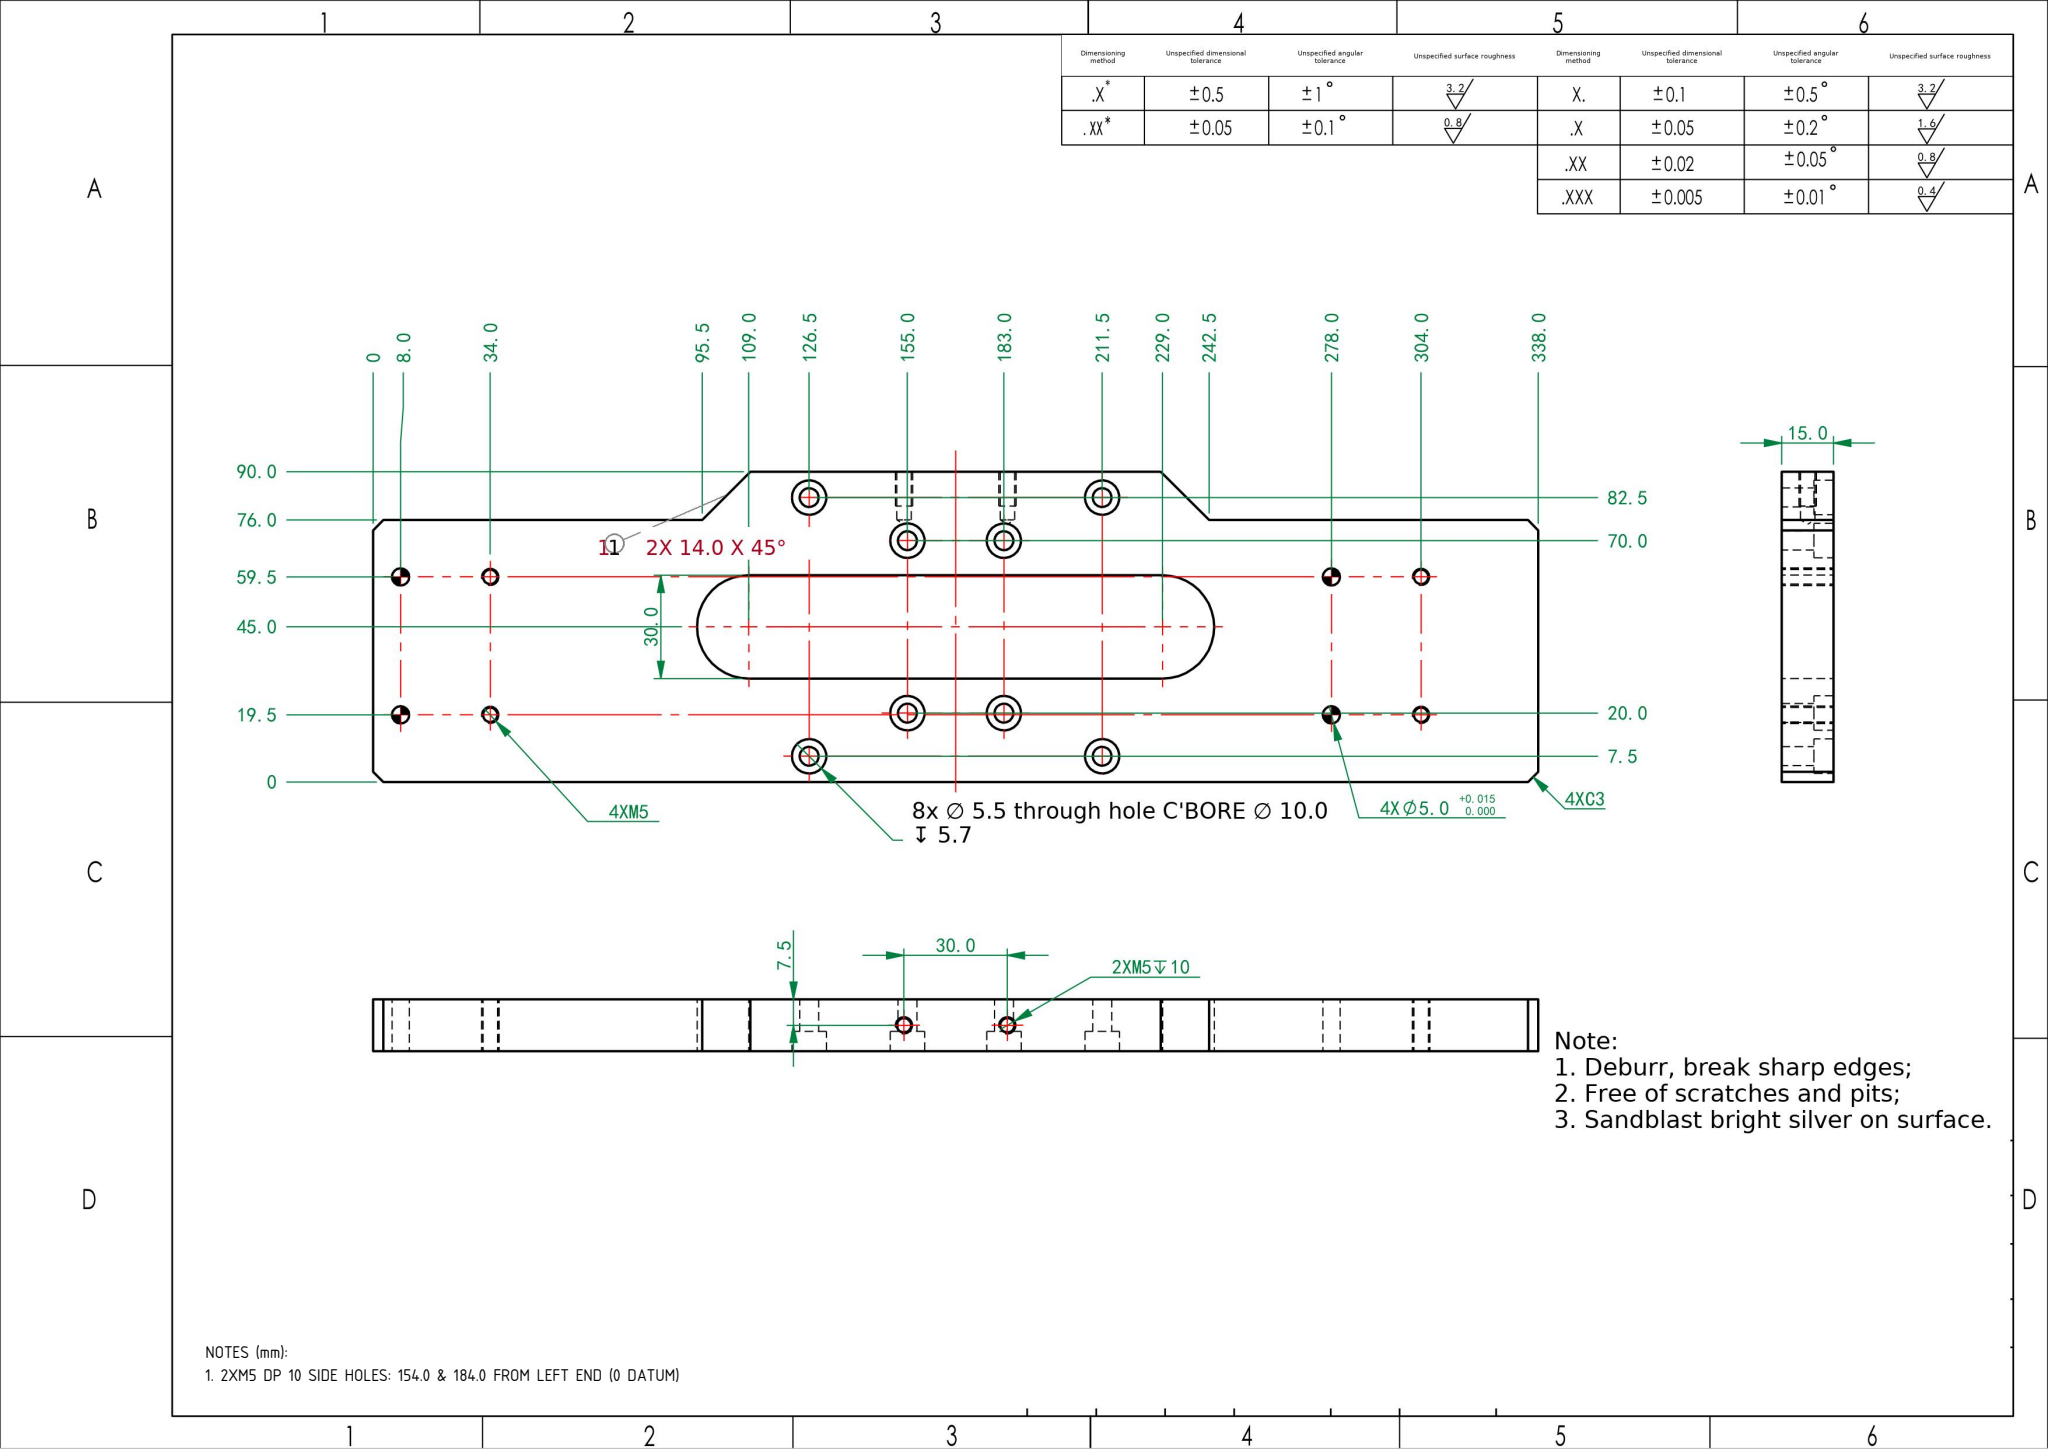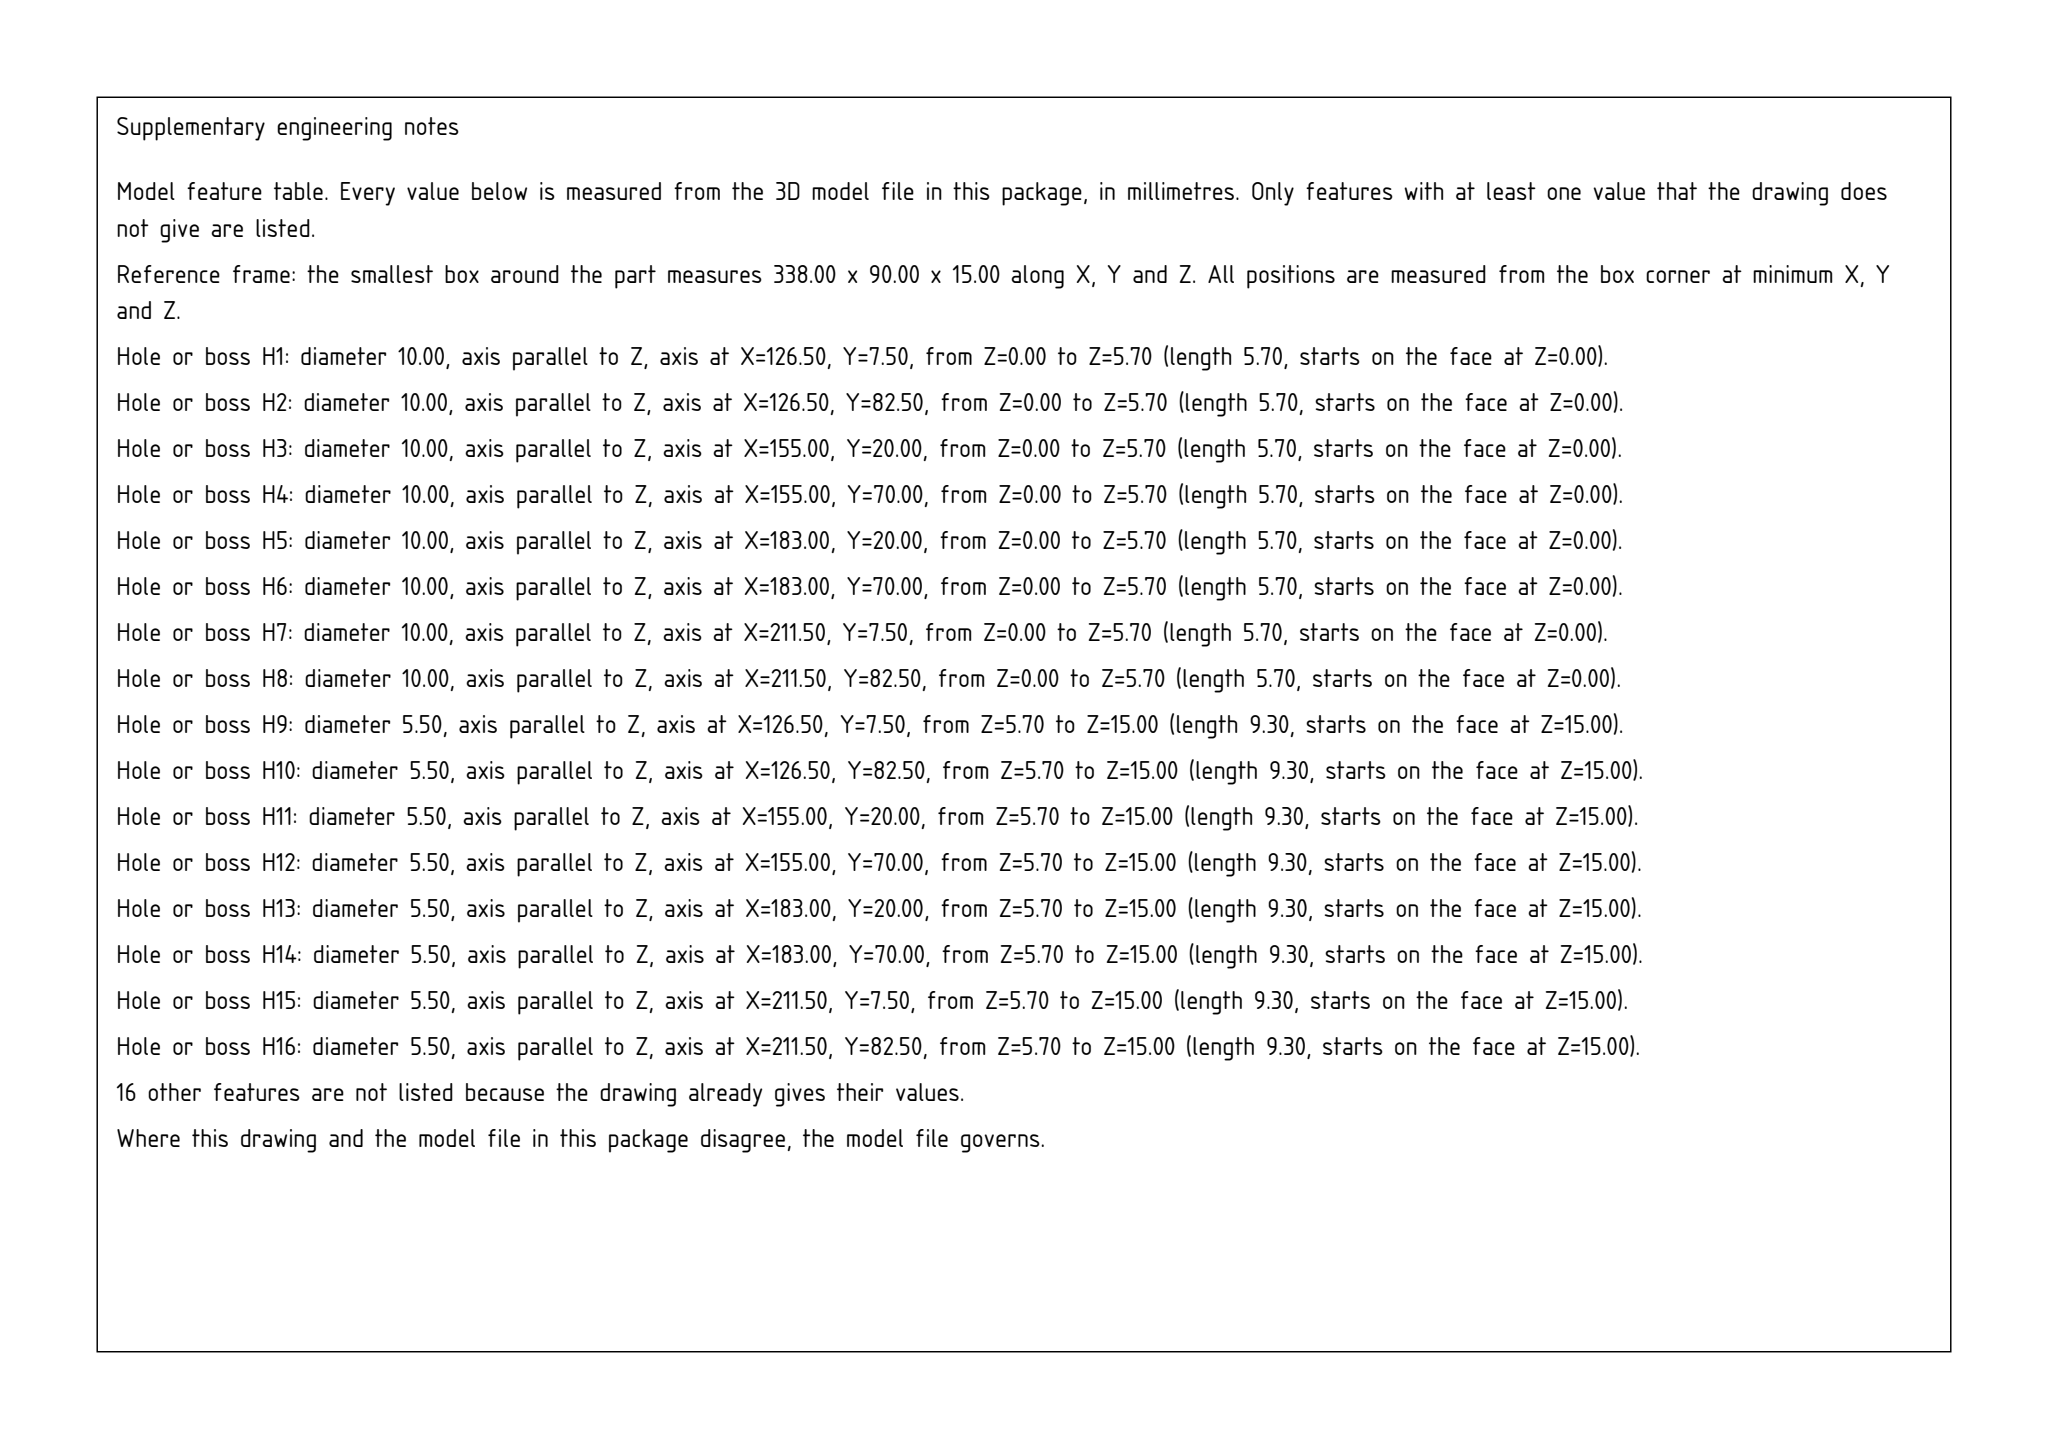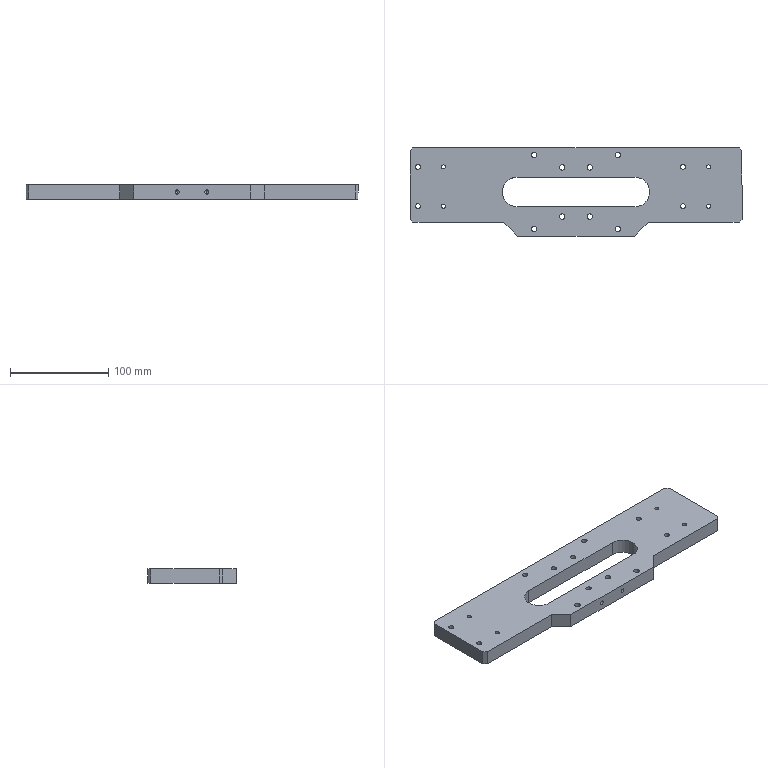Part | SolidWorks | mm | 1 solid | 83 faces | box 338 x 90 x 15 mm | volume 340619 mm3 | cylinder 55 | plane 24 | cone 4 | commonest cylinder face diameters 10 x16 5.5 x16 4.2 x12 5 x8 30 x3
Drawing notes:
2XM5 DP 10 SIDE HOLES: 154.0 & 184.0 FROM LEFT END (0 DATUM) | from the solid: cyl dia 4.2 axis y at x=154.0 and x=184.0, z=7.5, len 14.0; bbox x 0-338